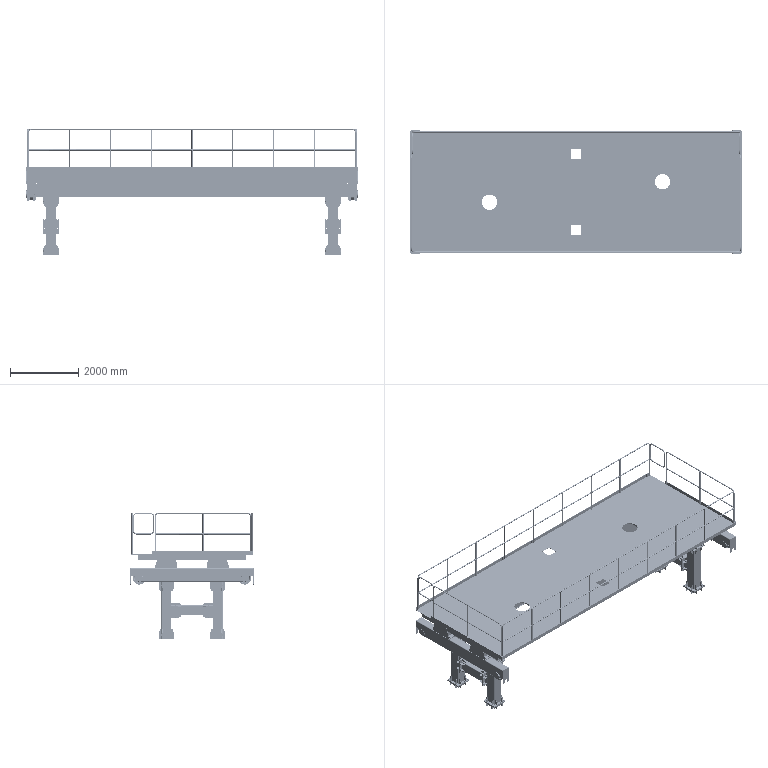Assembly | SolidWorks | mm | 353 component files | 557 solids | 9634 faces | box 9711 x 3600 x 3701.75 mm | volume 1285155719 mm3 | plane 4450 | cylinder 3136 | cone 1736 | torus 312 | commonest cylinder face diameters 21 x576 11 x384 12 x240 25 x192 20 x160 13 x144 24 x144 30 x128
Bill of materials:
Block | 24 | Plain Carbon Steel | Thin, flat square plate with rounded corners and no holes.
CrossRib | 2 |  | Multi-body fabricated frame: a long square hollow section with a bolted plate frame at each end, tapered gusset plates and protruding fin plates.
Door | 2 | Plain Carbon Steel | Closed loop of round-section rod or wire shaped as a square with large-radius rounded corners.
Flange10 | 4 | Plain Carbon Steel | Thin rectangular flat plate with sharp corners and two pairs of through-holes, one pair near each short end.
Flange20 | 4 | Plain Carbon Steel | Rectangular flat plate with sharp corners and a column of four through-holes along each short edge, eight holes in total.
GuardrailMountingPlate | 24 | Plain Carbon Steel | Thick rectangular plate with sharp corners and four through-holes, one near each corner.
Kick1 | 2 | Plain Carbon Steel | Very thin, flat rectangular sheet or strip that looks almost like a line in several views.
Kick2 | 2 | Plain Carbon Steel | Long, slender flat bar with small through-holes in groups of four at each end and at mid-length.
Link1 | 12 | Plain Carbon Steel | Long square hollow section with rounded corners and open ends. There is a slight offset or step at the ends.
Link2 | 24 | Plain Carbon Steel | Square hollow section with rounded corners and open ends, shorter relative to its cross-section than the similar tube body. There is a slight step at the ends.
350X125X10 | 8 | Plain Carbon Steel | Flat plate with a tapered profile, like a gusset: one long straight edge, one sloped edge, and a short straight section at the wide end.
650X450X360X10 | 4 | Plain Carbon Steel | Thin flat plate with a symmetric trapezoidal profile and short straight edges on each side at the wide base.
750X388X6 | 26 | Plain Carbon Steel | Thin flat rectangular plate with two narrow straight slots, one cut in from each long edge at about mid-height.
9340X450X10 | 2 | Plain Carbon Steel | Long, narrow, thin flat rectangular strip with no visible holes or features.
9340X60X6 | 4 | Plain Carbon Steel | Long, slender flat bar or strip with a thin rectangular cross-section and no visible features.
9940X450X10 | 2 | Plain Carbon Steel | Long, narrow, thin flat rectangular strip with no visible holes or features.
9940X9340X750X6 | 4 | Plain Carbon Steel | Long, thin flat bar with a stepped profile: a full-length upper band over a slightly shorter lower band, which leaves a shoulder notch at each end.
L | 4 | Plain Carbon Steel | Sheet bracket bent to a 90-degree L with a rounded inside bend. Both flanges have round through-holes near their ends.
Platform | 1 | Plain Carbon Steel | Very thin flat rectangular plate with two round holes and two small square holes.
PlatformGuardrail1 | 2 | Plain Carbon Steel | Slender round rod or wire bent into a wide U (staple-like shape) with rounded bends and two short parallel legs.
PlatformGuardrail2 | 16 | Plain Carbon Steel | Straight hollow round tube with plain cut ends.
PlatformGuardrail3 | 2 | Plain Carbon Steel | Long, slender straight hollow round tube with small evenly spaced marks along its length.
PlatformGuardrail4 | 2 | Plain Carbon Steel | Round rod or tube bent into a U shape with rounded bends and two longer parallel legs.
PlatformGuardrail5 | 2 | Plain Carbon Steel | Straight hollow round tube with a small circumferential groove or break at mid-length.
50 x 30 x 2.6x250 | 2 | Plain Carbon Steel | Long, straight, thin-walled hollow profile. The cross-section looks like a rectangle with rounded corners. Near each end, one side of the profile is cut back so the end sections are open channels (U-shaped). There is a rounded, roughly semicircular notch at each place where the cut-back ends meet the full-depth middle section.
380X230X6 | 8 | Plain Carbon Steel | Thin flat rectangular plate with four rounded corners and no visible holes or cutouts.
Finishing | 4 | Plain Carbon Steel | Thin flat rectangular plate with rounded outer corners, five round through-holes and a rectangular notch open to one short edge.
L756AngleBoxSingleEdgeWheelSet350-C | 4 |  | Axisymmetric wheel-like body with a single flange on one side. A short cylindrical housing projects from each face and has a ring of hex-head fasteners and a small central nipple-like protrusion.
100X75X8 | 64 | Plain Carbon Steel | Solid rectangular block (thick plate) with sharp edges and no visible features.
150X75X8 | 64 | Plain Carbon Steel | Flat plate of uniform thickness with an irregular five-sided outline: two parallel vertical edges of different heights, a short flat top, a long angled edge and a straight bottom edge.
300 x 300 x 8-100 | 8 | Plain Carbon Steel | Short, thin-walled square tube section (open frame ring) with rounded outer and inner corners, open at both ends.
300 x 300 x 8-1200 | 4 | Plain Carbon Steel | Long, thin-walled square hollow tube with rounded corners and open, square-cut ends.
450X450X20 | 16 | Plain Carbon Steel | Thin flat square plate with rounded corners and twelve round through-holes evenly spaced around the edge, four per side including the corners.
Mates:
1. coincident | Main-1/9940X450X10-1 face at (-3372.199, 2146.323, 5575.973) dir (0, 0, 1) | Platform-1 face at (1462.801, 1171.323, 5575.973) dir (0, 0, -1)
2. coincident | Main-2/650X450X360X10-2 face at (6307.801, 746.323, 5575.973) dir (1, 0, 0) | Platform-1 face at (6307.801, 2961.323, 5575.973) dir (1, 0, 0)
3. coincident | Platform-1 edge at (-3382.199, 1171.323, 5575.973) dir (1, 0, 0) | assembly plane at (0, 1171.323, 0) dir (0, -1, 0)
4. coincident | Main-1/L-1 face at (-3392.199, 1596.323, 5195.973) dir (0, 0, -1) | Flange10-1 face at (-3392.199, 1596.323, 5195.973) dir (0, 0, 1)
5. concentric | Main-1/L-1 face at (-3307.199, 2196.323, 4795.973) dir (0, 0, 1) r 12.5 | Flange10-1 face at (-3307.199, 2196.323, 4775.973) dir (0, 0, 1) r 12.5
6. concentric | Main-1/L-1 face at (-3307.199, 1646.323, 4795.973) dir (0, 0, 1) r 12.5 | Flange10-1 face at (-3307.199, 1646.323, 4775.973) dir (0, 0, 1) r 12.5
7. coincident | Main-1/L-1 face at (-3092.199, 1596.323, 5215.973) dir (-1, 0, 0) | Flange20-1 face at (-3092.199, 2246.323, 5215.973) dir (1, 0, 0)
8. concentric | Main-1/L-1 face at (-3392.199, 2196.323, 4870.973) dir (1, 0, 0) r 12.5 | Flange20-1 face at (-2792.199, 2196.323, 4870.973) dir (-1, 0, 0) r 12.5
9. concentric | Main-1/L-1 face at (-3392.199, 1646.323, 5140.973) dir (1, 0, 0) r 12.5 | Flange20-1 face at (-2792.199, 1646.323, 5140.973) dir (-1, 0, 0) r 12.5
10. coincident | Flange20-2 face at (-3112.199, 746.323, 5215.973) dir (-1, 0, 0) | Short-1/3650-1 face at (-3112.199, -618.677, 5165.973) dir (1, 0, 0)
11. coincident | Flange10-1 face at (-3392.199, 1596.323, 5185.973) dir (0, 0, -1) | Short-1/3650-1 face at (-3132.199, -618.677, 5185.973) dir (0, 0, 1)
12. coincident | Short-1 plane at (-2112.199, 1171.323, 4760.606) dir (0, 1, 0) | assembly plane at (0, 1171.323, 0) dir (0, -1, 0)
13. coincident | Flange20-4 face at (6037.801, 746.323, 5215.973) dir (1, 0, 0) | Short-3/3650-1 face at (6037.801, 2961.323, 5165.973) dir (-1, 0, 0)
14. coincident | Flange10-4 face at (6317.801, 746.323, 5185.973) dir (0, 0, -1) | Short-3/3650-1 face at (6057.801, 2961.323, 5185.973) dir (0, 0, 1)
15. coincident | Short-1/Finishing-1 face at (-3197.199, -628.677, 4795.973) dir (0, -1, 0) | Short-3/Finishing-2 face at (6202.801, -628.677, 4795.973) dir (0, -1, 0)
16. coincident | Main-1/9340X450X10-1 face at (-3072.199, 2146.323, 4805.973) dir (0, 0, -1) | TrolleyLeg-1/300 x 300 x 8-100-1 face at (-2796.199, 2055.323, 4805.973) dir (0, 0, 1)
17. coincident | Main-1/9340X450X10-1 face at (-3072.199, 2146.323, 4805.973) dir (0, 1, 0) | TrolleyLeg-1/450X450X20-3 face at (-2872.199, 2146.323, 4685.973) dir (0, 1, 0)
18. distance | assembly plane at (1462.801, 0, 0) dir (-1, 0, 0) | TrolleyLeg-1/300 x 300 x 8-100-1 edge at (-2662.199, 2071.323, 4805.973) dir (1, 0, 0)
19. coincident | TrolleyLeg-2/300 x 300 x 8-1200-1 face at (5737.801, 1787.323, 3245.973) dir (1, 0, 0) | CrossRib-1 face at (5737.801, 711.323, 4089.973) dir (1, 0, 0)
20. coincident | TrolleyLeg-2/300 x 300 x 8-1200-1 face at (5721.801, 1771.323, 3245.973) dir (0, -1, 0) | CrossRib-1 face at (5453.801, 1771.323, 3821.973) dir (0, 1, 0)
21. distance | CrossRib-1 face at (5453.801, 711.323, 3805.973) dir (0, 0, -1) | TrolleyLeg-2/300 x 300 x 8-100-2 face at (5721.801, 1787.323, 3105.973) dir (0, 0, -1)
22. coincident | Platform-1 face at (1462.801, 1171.323, 5585.973) dir (0, 0, 1) | Kick1-1 face at (-3382.199, 2951.323, 5585.973) dir (0, 0, -1)
23. parallel | Platform-1 face at (-3382.199, 2961.323, 5575.973) dir (0, 1, 0) | Kick1-1 face at (-3382.199, 2961.323, 5585.973) dir (0, 1, 0)
24. coincident | Platform-1 face at (6307.801, 2961.323, 5575.973) dir (1, 0, 0) | Kick1-1 face at (6307.801, 2951.323, 5585.973) dir (1, 0, 0)
25. coincident | Platform-1 face at (1462.801, 1171.323, 5585.973) dir (0, 0, 1) | Kick2-1 face at (6307.801, -608.677, 5585.973) dir (0, 0, -1)
26. distance | Kick1-1 face at (-3382.199, 2951.323, 5585.973) dir (0, -1, 0) | Platform-1 face at (-3382.199, 2961.323, 5575.973) dir (0, 1, 0)
27. coincident | Platform-1 face at (6307.801, 2961.323, 5575.973) dir (1, 0, 0) | Kick2-1 face at (6307.801, -608.677, 5585.973) dir (1, 0, 0)
28. coincident | Platform-1 face at (1462.801, 1171.323, 5575.973) dir (0, 0, -1) | Link1-1 face at (4455.801, 621.323, 5575.973) dir (0, 0, 1)
29. coincident | Main-2/9940X9340X750X6-1 face at (-3372.199, 621.323, 5565.973) dir (0, 1, 0) | Link1-1 face at (4455.801, 621.323, 5563.973) dir (0, -1, 0)
30. distance | Link1-1 face at (4317.801, 621.323, 5437.973) dir (-1, 0, 0) | Platform-1 face at (3992.801, 1471.323, 5575.973) dir (0, 0, 1) r 225
31. coincident | Main-2/9940X9340X750X6-2 face at (-3372.199, 221.323, 5565.973) dir (0, -1, 0) | Link2-1 edge at (4467.801, 221.323, 5563.973) dir (0, 0, -1)
32. coincident | Platform-1 face at (1462.801, 1171.323, 5575.973) dir (0, 0, -1) | Link2-1 face at (4455.801, -393.677, 5575.973) dir (0, 0, 1)
33. coincident | Link1-1 face at (4467.801, 621.323, 5563.973) dir (1, 0, 0) | Link2-1 face at (4467.801, -393.677, 5563.973) dir (1, 0, 0)
34. coincident | Platform-1 face at (1462.801, 1171.323, 5575.973) dir (0, 0, -1) | Link2-13 face at (4329.801, 2736.323, 5575.973) dir (0, 0, 1)
35. coincident | Main-1/9940X9340X750X6-1 face at (-3372.199, 2121.323, 5565.973) dir (0, 1, 0) | Link2-13 edge at (4467.801, 2121.323, 5500.973) dir (1, 0, 0)
36. coincident | Link1-1 face at (4317.801, 621.323, 5437.973) dir (-1, 0, 0) | Link2-13 face at (4317.801, 2736.323, 5563.973) dir (-1, 0, 0)
37. coincident | Link2-13 face at (4329.801, 2736.323, 5563.973) dir (0, 1, 0) | Block-1 face at (4333.801, 2736.323, 5559.973) dir (0, 1, 0)
38. coincident | Link2-13 face at (4461.801, 2736.323, 5437.973) dir (-1, 0, 0) | Block-1 face at (4461.801, 2730.323, 5441.973) dir (1, 0, 0)
39. coincident | Link2-13 face at (4455.801, 2736.323, 5431.973) dir (0, 0, 1) | Block-1 face at (4333.801, 2730.323, 5431.973) dir (0, 0, -1)
40. coincident | Link2-1 face at (4455.801, -393.677, 5563.973) dir (0, -1, 0) | Block-15 face at (4333.801, -393.677, 5559.973) dir (0, -1, 0)
41. coincident | Link2-1 face at (4323.801, -393.677, 5437.973) dir (1, 0, 0) | Block-15 face at (4323.801, -393.677, 5441.973) dir (-1, 0, 0)
42. coincident | Link2-1 face at (4329.801, -393.677, 5431.973) dir (0, 0, 1) | Block-15 face at (4333.801, -393.677, 5431.973) dir (0, 0, -1)
43. distance | Platform-1 face at (1462.801, 1171.323, 5585.973) dir (0, 0, 1) | PlatformGuardrail1-1 face at (-3322.199, -581.927, 5590.973) dir (0, 0, -1)
44. coincident | Kick1-2 face at (-3382.199, -608.677, 5685.973) dir (0, 1, 0) | GuardrailMountingPlate-1 face at (-3372.199, -608.677, 5585.973) dir (0, -1, 0)
45. coincident | Platform-1 face at (1462.801, 1171.323, 5585.973) dir (0, 0, 1) | GuardrailMountingPlate-1 face at (-3372.199, -608.677, 5585.973) dir (0, 0, -1)
46. coincident | Kick2-2 face at (-3372.199, -608.677, 5685.973) dir (1, 0, 0) | GuardrailMountingPlate-1 face at (-3372.199, -608.677, 5585.973) dir (-1, 0, 0)
47. distance | PlatformGuardrail1-1 face at (-3322.199, -581.927, 6690.973) dir (0, 0, -1) r 13.75 | GuardrailMountingPlate-1 face at (-3372.199, -598.677, 5585.973) dir (0, 1, 0)
48. distance | PlatformGuardrail1-1 face at (-3322.199, -581.927, 6690.973) dir (0, 0, -1) r 13.75 | GuardrailMountingPlate-1 face at (-3372.199, -608.677, 5585.973) dir (-1, 0, 0)
49. distance | GuardrailMountingPlate-1 face at (-3372.199, -598.677, 5585.973) dir (0, 1, 0) | PlatformGuardrail1-1 face at (6247.801, -581.927, 5590.973) dir (0, 0, 1) r 13.75
50. distance | PlatformGuardrail2-1 face at (-2110.949, -581.927, 6774.223) dir (0, 0, -1) r 16.75 | GuardrailMountingPlate-2 face at (-2180.949, -598.677, 5585.973) dir (0, 1, 0)
51. distance | GuardrailMountingPlate-2 face at (-2180.949, -608.677, 5585.973) dir (-1, 0, 0) | PlatformGuardrail2-1 face at (-2110.949, -581.927, 6774.223) dir (0, 0, -1) r 16.75
52. distance | PlatformGuardrail2-1 face at (-2110.949, -581.927, 6774.223) dir (0, 0, 1) | PlatformGuardrail1-1 face at (6147.801, -581.927, 6790.973) dir (-1, 0, 0) r 13.75
53. distance | Platform-1 face at (1462.801, 1171.323, 5585.973) dir (0, 0, 1) | PlatformGuardrail3-1 face at (-3305.449, -581.927, 6185.973) dir (1, 0, 0) r 16.75
54. distance | GuardrailMountingPlate-2 face at (-2180.949, -598.677, 5585.973) dir (0, 1, 0) | PlatformGuardrail3-1 face at (-3305.449, -581.927, 6185.973) dir (1, 0, 0) r 16.75
55. distance | PlatformGuardrail1-1 face at (-3322.199, -581.927, 6690.973) dir (0, 0, -1) r 13.75 | PlatformGuardrail3-1 face at (-3305.449, -581.927, 6185.973) dir (-1, 0, 0)
56. coincident | Kick2-1 face at (6297.801, -608.677, 5585.973) dir (-1, 0, 0) | GuardrailMountingPlate-19 face at (6297.801, -598.677, 5585.973) dir (1, 0, 0)
57. coincident | Kick2-1 face at (6307.801, -608.677, 5685.973) dir (0, 0, 1) | GuardrailMountingPlate-19 face at (6297.801, -598.677, 5685.973) dir (0, 0, 1)
58. coincident | GuardrailMountingPlate-9 face at (6157.801, -598.677, 5585.973) dir (0, 1, 0) | GuardrailMountingPlate-19 face at (6297.801, -598.677, 5585.973) dir (0, -1, 0)
59. distance | PlatformGuardrail4-1 face at (6271.051, -551.927, 5590.973) dir (0, 0, -1) | Platform-1 face at (1462.801, 1171.323, 5585.973) dir (0, 0, 1)
60. distance | GuardrailMountingPlate-19 face at (6287.801, -598.677, 5585.973) dir (-1, 0, 0) | PlatformGuardrail4-1 face at (6271.051, -551.927, 5590.973) dir (0, 0, 1) r 16.75
61. distance | PlatformGuardrail4-1 face at (6271.051, -551.927, 5590.973) dir (0, 0, 1) r 16.75 | Kick1-2 face at (-3382.199, -608.677, 5685.973) dir (0, 1, 0)
62. coincident | Kick2-1 face at (6297.801, -608.677, 5585.973) dir (-1, 0, 0) | GuardrailMountingPlate-20 face at (6297.801, 2194.823, 5585.973) dir (1, 0, 0)
63. coincident | Kick2-1 face at (6307.801, -608.677, 5685.973) dir (0, 0, 1) | GuardrailMountingPlate-20 face at (6297.801, 2194.823, 5685.973) dir (0, 0, 1)
64. distance | PlatformGuardrail4-1 face at (6271.051, 2248.073, 6690.973) dir (0, 0, -1) r 16.75 | GuardrailMountingPlate-20 face at (6297.801, 2334.823, 5585.973) dir (0, 1, 0)
65. distance | GuardrailMountingPlate-21 face at (6287.801, 794.823, 5585.973) dir (-1, 0, 0) | PlatformGuardrail2-15 face at (6271.051, 848.073, 6774.223) dir (0, 0, -1) r 16.75
66. coincident | PlatformGuardrail2-7 face at (5036.551, -581.927, 6774.223) dir (0, 0, 1) | PlatformGuardrail2-15 face at (6271.051, 848.073, 6774.223) dir (0, 0, 1)
67. distance | PlatformGuardrail2-15 face at (6271.051, 848.073, 6774.223) dir (0, 0, -1) r 16.75 | GuardrailMountingPlate-21 face at (6297.801, 934.823, 5585.973) dir (0, 1, 0)
68. distance | Platform-1 face at (1462.801, 1171.323, 5585.973) dir (0, 0, 1) | PlatformGuardrail5-1 face at (6271.051, 2224.823, 6185.973) dir (0, -1, 0) r 16.75
69. distance | GuardrailMountingPlate-21 face at (6287.801, 794.823, 5585.973) dir (-1, 0, 0) | PlatformGuardrail5-1 face at (6271.051, 2224.823, 6185.973) dir (0, -1, 0) r 16.75
70. distance | PlatformGuardrail4-1 face at (6271.051, -551.927, 5590.973) dir (0, 0, 1) r 16.75 | PlatformGuardrail5-1 face at (6271.051, -535.177, 6185.973) dir (0, -1, 0)
71. distance | Door-1 face at (6247.801, 2888.323, 6685.973) dir (0, 0, 1) r 16.75 | Kick2-1 face at (6297.801, -608.677, 5585.973) dir (-1, 0, 0)
72. distance | Door-1 face at (6247.801, 2888.323, 6685.973) dir (0, 0, 1) r 16.75 | Kick1-1 face at (-3382.199, 2961.323, 5585.973) dir (0, 1, 0)
73. distance | Door-1 face at (6247.801, 2788.323, 6185.973) dir (0, 1, 0) r 16.75 | Platform-1 face at (1462.801, 1171.323, 5585.973) dir (0, 0, 1)
74. coincident | 9940X450X10-1 face at (-6309.119, 904.191, 1000) dir (0, -1, 0) | 9940X9340X750X6-1 face at (-6309.119, 904.191, 1025) dir (0, 1, 0)
75. coincident | 9940X450X10-1 face at (-6309.119, 904.191, 1000) dir (-1, 0, 0) | 9940X9340X750X6-1 face at (-6309.119, 554.191, 1025) dir (-1, 0, 0)
76. distance | 9940X450X10-1 face at (-6309.119, 904.191, 1000) dir (0, 0, -1) | 9940X9340X750X6-1 face at (-6309.119, 904.191, 1025) dir (0, 0, -1)
77. coincident | 9940X9340X750X6-1 face at (-6309.119, 904.191, 1031) dir (0, 0, 1) | 750X388X6-1 face at (-5868.119, 154.191, 1031) dir (0, 0, -1)
78. coincident | 9940X450X10-1 face at (-6309.119, 904.191, 1000) dir (0, -1, 0) | 750X388X6-1 face at (-5868.119, 904.191, 1031) dir (0, 1, 0)
79. distance | 750X388X6-1 face at (-5874.119, 904.191, 1031) dir (-1, 0, 0) | 9940X9340X750X6-1 face at (-6009.119, 154.191, 1025) dir (-1, 0, 0)
80. coincident | 750X388X6-1 face at (-5868.119, 524.191, 1031) dir (0, 1, 0) | 9340X60X6-1 face at (-6009.119, 524.191, 1031) dir (0, -1, 0)
81. coincident | 9940X9340X750X6-1 face at (-6309.119, 904.191, 1031) dir (0, 0, 1) | 9340X60X6-1 face at (-6009.119, 524.191, 1031) dir (0, 0, -1)
82. coincident | 9940X9340X750X6-1 face at (-6009.119, 154.191, 1025) dir (-1, 0, 0) | 9340X60X6-1 face at (-6009.119, 524.191, 1031) dir (-1, 0, 0)
83. coincident | 750X388X6-1 face at (-5868.119, 524.191, 1354) dir (0, 1, 0) | 9340X60X6-2 face at (-6009.119, 524.191, 1359) dir (0, -1, 0)
84. coincident | 750X388X6-1 face at (-5868.119, 904.191, 1419) dir (0, 0, 1) | 9340X60X6-2 face at (-6009.119, 524.191, 1419) dir (0, 0, 1)
85. coincident | 9340X60X6-1 face at (-6009.119, 524.191, 1031) dir (-1, 0, 0) | 9340X60X6-2 face at (-6009.119, 524.191, 1359) dir (-1, 0, 0)
86. coincident | 750X388X6-1 face at (-5868.119, 154.191, 1419) dir (0, -1, 0) | 9340X450X10-1 face at (-6009.119, 154.191, 1000) dir (0, 1, 0)
87. coincident | 9940X450X10-1 face at (-6309.119, 904.191, 1000) dir (0, 0, -1) | 9340X450X10-1 face at (-6009.119, 144.191, 1000) dir (0, 0, -1)
88. coincident | 9940X9340X750X6-1 face at (-6009.119, 154.191, 1025) dir (-1, 0, 0) | 9340X450X10-1 face at (-6009.119, 144.191, 1000) dir (-1, 0, 0)
89. coincident | 750X388X6-1 face at (-5868.119, 524.191, 1419) dir (0, 0, 1) | 9940X9340X750X6-2 face at (-6309.119, 904.191, 1419) dir (0, 0, -1)
90. coincident | 9940X450X10-1 face at (-6309.119, 904.191, 1000) dir (0, -1, 0) | 9940X9340X750X6-2 face at (-6309.119, 904.191, 1419) dir (0, 1, 0)
91. coincident | 9940X450X10-1 face at (-6309.119, 904.191, 1000) dir (-1, 0, 0) | 9940X9340X750X6-2 face at (-6309.119, 554.191, 1419) dir (-1, 0, 0)
92. coincident | 9940X9340X750X6-2 face at (-6009.119, 154.191, 1419) dir (-1, 0, 0) | L-1 face at (-6009.119, 554.191, 1550) dir (1, 0, 0)
93. coincident | 9940X9340X750X6-2 face at (-6009.119, 554.191, 1419) dir (0, -1, 0) | L-1 face at (-6329.119, 554.191, 1550) dir (0, 1, 0)
94. distance | 9940X9340X750X6-1 face at (-6309.119, 904.191, 1025) dir (0, 0, -1) | L-1 face at (-6029.119, 509.191, 900) dir (0, 0, -1)
95. coincident | 9940X9340X750X6-2 face at (-6309.119, 554.191, 1419) dir (-1, 0, 0) | 650X450X360X10-1 face at (-6309.119, 914.191, 1550) dir (1, 0, 0)
96. coincident | L-1 face at (-6329.119, 554.191, 1550) dir (0, 1, 0) | 650X450X360X10-1 face at (-6319.119, 554.191, 900) dir (0, -1, 0)
97. coincident | L-1 face at (-6054.119, 509.191, 1550) dir (0, 0, 1) | 650X450X360X10-1 face at (-6319.119, 554.191, 1550) dir (0, 0, 1)
98. coincident | L-1 face at (-6054.119, 509.191, 1550) dir (0, 0, 1) | 350X125X10-1 face at (-6054.119, 604.191, 1550) dir (0, 0, 1)
99. coincident | L-1 edge at (-6054.119, 554.191, 1550) dir (0, 0, -1) | 350X125X10-1 edge at (-6054.119, 554.191, 1425) dir (0, 0, 1)
100. coincident | L-1 face at (-6329.119, 554.191, 1550) dir (0, 1, 0) | 350X125X10-1 face at (-6054.119, 554.191, 1550) dir (0, -1, 0)
101. coincident | L-1 face at (-6029.119, 509.191, 900) dir (0, 0, -1) | 350X125X10-2 face at (-6064.119, 604.191, 900) dir (0, 0, -1)
102. coincident | L-1 edge at (-6054.119, 554.191, 1550) dir (0, 0, -1) | 350X125X10-2 face at (-6064.119, 554.191, 900) dir (0, -1, 0)
103. coincident | L-1 edge at (-6054.119, 554.191, 1550) dir (0, 0, -1) | 350X125X10-2 face at (-6054.119, 904.191, 1025) dir (1, 0, 0)
104. coincident | L-1 face at (-6329.119, 554.191, 1550) dir (0, 1, 0) | 350X125X10-2 face at (-6064.119, 554.191, 900) dir (0, -1, 0)
105. distance | 380X230X6-1 face at (-3007.575, 400.367, 1025) dir (-1, 0, 0) | 3650-1 face at (-3622.575, 45.367, 1230) dir (-1, 0, 0)
106. coincident | 3650-1 face at (-42.575, 415.367, 1020) dir (0, -1, 0) | 380X230X6-1 face at (-2997.575, 415.367, 1025) dir (0, 1, 0)
107. coincident | 3650-1 face at (-42.575, 405.367, 1010) dir (0, 0, 1) | 380X230X6-1 face at (-2997.575, 50.367, 1010) dir (0, 0, -1)
108. concentric | 3650-1 face at (-3372.575, 135.367, 1250) dir (0, 0, -1) r 105 | L756AngleBoxSingleEdgeWheelSet350-C-3 face at (-3372.575, 135.367, 1060) dir (0, 0, -1) r 105
109. distance | L756AngleBoxSingleEdgeWheelSet350-C-3 face at (-3402.058, 209.737, 979.5) dir (0, 0, -1) | 3650-1 face at (-42.575, 405.367, 1000) dir (0, 0, -1)
110. concentric | 3650-1 face at (-292.575, 135.367, 1250) dir (0, 0, -1) r 105 | L756AngleBoxSingleEdgeWheelSet350-C-4 face at (-292.575, 135.367, 1060) dir (0, 0, -1) r 105
111. distance | L756AngleBoxSingleEdgeWheelSet350-C-4 face at (-322.058, 209.737, 979.5) dir (0, 0, -1) | 3650-1 face at (-42.575, 405.367, 1000) dir (0, 0, -1)
112. coincident | 3650-1 face at (-42.575, 45.367, 1230) dir (1, 0, 0) | Finishing-1 face at (-42.575, 35.367, 1085) dir (-1, 0, 0)
113. coincident | 3650-1 face at (-42.575, 45.367, 1250) dir (0, 0, 1) | Finishing-1 face at (-32.575, 415.367, 1250) dir (0, 0, 1)
114. coincident | 3650-1 face at (-42.575, 425.367, 1020) dir (0, 1, 0) | Finishing-1 face at (-32.575, 425.367, 1010) dir (0, 1, 0)
115. coincident | 450X450X20-1 face at (1257.496, 982.157, 1230.34) dir (0, 1, 0) | 300 x 300 x 8-1200-1 face at (913.496, 982.157, 1306.34) dir (0, -1, 0)
116. distance | 300 x 300 x 8-1200-1 face at (897.496, 982.157, 1306.34) dir (-1, 0, 0) | 450X450X20-1 face at (822.496, 962.157, 1230.34) dir (-1, 0, 0)
117. distance | 300 x 300 x 8-1200-1 face at (913.496, 982.157, 1290.34) dir (0, 0, -1) | 450X450X20-1 face at (837.496, 962.157, 1215.34) dir (0, 0, -1)
118. coincident | 300 x 300 x 8-1200-1 face at (913.496, 2402.157, 1306.34) dir (0, 1, 0) | 450X450X20-2 face at (1257.496, 2402.157, 1230.34) dir (0, -1, 0)
119. distance | 300 x 300 x 8-1200-1 face at (913.496, 982.157, 1290.34) dir (0, 0, -1) | 450X450X20-2 face at (837.496, 2402.157, 1215.34) dir (0, 0, -1)
120. distance | 450X450X20-2 face at (822.496, 2402.157, 1230.34) dir (-1, 0, 0) | 300 x 300 x 8-1200-1 face at (897.496, 982.157, 1306.34) dir (-1, 0, 0)
121. coincident | 450X450X20-2 face at (1257.496, 2422.157, 1230.34) dir (0, 1, 0) | 450X450X20-3 face at (1257.496, 2422.157, 1230.34) dir (0, -1, 0)
122. concentric | 450X450X20-2 face at (852.496, 2402.157, 1635.34) dir (0, 1, 0) r 10.5 | 450X450X20-3 face at (852.496, 2422.157, 1635.34) dir (0, 1, 0) r 10.5
123. concentric | 450X450X20-2 face at (1242.496, 2402.157, 1245.34) dir (0, 1, 0) r 10.5 | 450X450X20-3 face at (1242.496, 2422.157, 1245.34) dir (0, 1, 0) r 10.5
124. coincident | 450X450X20-3 face at (1257.496, 2442.157, 1230.34) dir (0, 1, 0) | 300 x 300 x 8-100-1 face at (913.496, 2442.157, 1306.34) dir (0, -1, 0)
125. coincident | 300 x 300 x 8-1200-1 face at (897.496, 982.157, 1306.34) dir (-1, 0, 0) | 300 x 300 x 8-100-1 face at (897.496, 2442.157, 1306.34) dir (-1, 0, 0)
126. coincident | 300 x 300 x 8-1200-1 face at (913.496, 982.157, 1290.34) dir (0, 0, -1) | 300 x 300 x 8-100-1 face at (913.496, 2442.157, 1290.34) dir (0, 0, -1)
127. coincident | 300 x 300 x 8-100-1 face at (897.496, 2442.157, 1306.34) dir (-1, 0, 0) | 100X75X8-1 face at (897.496, 2542.157, 1326.34) dir (1, 0, 0)
128. coincident | 300 x 300 x 8-100-1 face at (913.496, 2542.157, 1306.34) dir (0, 1, 0) | 100X75X8-1 face at (822.496, 2542.157, 1326.34) dir (0, 1, 0)
129. distance | 450X450X20-3 face at (837.496, 2422.157, 1215.34) dir (0, 0, -1) | 100X75X8-1 face at (822.496, 2542.157, 1326.34) dir (0, 0, -1)
130. coincident | 300 x 300 x 8-100-1 face at (897.496, 2442.157, 1306.34) dir (-1, 0, 0) | 100X75X8-2 face at (897.496, 2542.157, 1544.34) dir (1, 0, 0)
131. coincident | 300 x 300 x 8-100-1 face at (913.496, 2542.157, 1306.34) dir (0, 1, 0) | 100X75X8-2 face at (822.496, 2542.157, 1544.34) dir (0, 1, 0)
132. distance | 300 x 300 x 8-100-1 face at (1181.496, 2442.157, 1590.34) dir (0, 0, 1) | 100X75X8-2 face at (822.496, 2542.157, 1554.34) dir (0, 0, 1)
133. coincident | 450X450X20-3 face at (837.496, 2422.157, 1665.34) dir (0, 0, 1) | 100X75X8-3 face at (933.496, 2542.157, 1665.34) dir (0, 0, 1)
134. coincident | 300 x 300 x 8-100-1 face at (913.496, 2542.157, 1306.34) dir (0, 1, 0) | 100X75X8-3 face at (933.496, 2542.157, 1665.34) dir (0, 1, 0)
135. distance | 300 x 300 x 8-100-1 face at (897.496, 2442.157, 1306.34) dir (-1, 0, 0) | 100X75X8-3 face at (933.496, 2542.157, 1665.34) dir (-1, 0, 0)
136. coincident | 300 x 300 x 8-100-1 face at (913.496, 2542.157, 1306.34) dir (0, 1, 0) | 100X75X8-4 face at (1151.496, 2542.157, 1665.34) dir (0, 1, 0)
137. coincident | 450X450X20-3 face at (837.496, 2422.157, 1665.34) dir (0, 0, 1) | 100X75X8-4 face at (1151.496, 2542.157, 1665.34) dir (0, 0, 1)
138. distance | 300 x 300 x 8-100-1 face at (1197.496, 2442.157, 1574.34) dir (1, 0, 0) | 100X75X8-4 face at (1161.496, 2542.157, 1665.34) dir (1, 0, 0)
139. coincident | 450X450X20-1 face at (1257.496, 982.157, 1230.34) dir (0, 1, 0) | 150X75X8-1 face at (1153.496, 982.157, 1215.34) dir (0, -1, 0)
140. coincident | 450X450X20-1 face at (837.496, 962.157, 1215.34) dir (0, 0, -1) | 150X75X8-1 face at (1153.496, 1032.157, 1215.34) dir (0, 0, -1)
141. distance | 300 x 300 x 8-1200-1 face at (1197.496, 982.157, 1574.34) dir (1, 0, 0) | 150X75X8-1 face at (1161.496, 1132.157, 1290.34) dir (1, 0, 0)
142. coincident | 450X450X20-1 face at (1257.496, 982.157, 1230.34) dir (0, 1, 0) | 150X75X8-2 face at (933.496, 982.157, 1215.34) dir (0, -1, 0)
143. coincident | 450X450X20-1 face at (837.496, 962.157, 1215.34) dir (0, 0, -1) | 150X75X8-2 face at (933.496, 1032.157, 1215.34) dir (0, 0, -1)
144. distance | 300 x 300 x 8-1200-1 face at (897.496, 982.157, 1306.34) dir (-1, 0, 0) | 150X75X8-2 face at (933.496, 1132.157, 1290.34) dir (-1, 0, 0)
145. coincident | 450X450X20-1 face at (1257.496, 982.157, 1230.34) dir (0, 1, 0) | 150X75X8-3 face at (1272.496, 982.157, 1326.34) dir (0, -1, 0)
146. coincident | 450X450X20-1 face at (1272.496, 962.157, 1230.34) dir (1, 0, 0) | 150X75X8-3 face at (1272.496, 1032.157, 1326.34) dir (1, 0, 0)
147. distance | 150X75X8-3 face at (1197.496, 1132.157, 1326.34) dir (0, 0, -1) | 300 x 300 x 8-1200-1 face at (913.496, 982.157, 1290.34) dir (0, 0, -1)
148. coincident | 450X450X20-1 face at (1257.496, 982.157, 1230.34) dir (0, 1, 0) | 150X75X8-4 face at (1272.496, 982.157, 1546.34) dir (0, -1, 0)
149. coincident | 450X450X20-1 face at (1272.496, 962.157, 1230.34) dir (1, 0, 0) | 150X75X8-4 face at (1272.496, 1032.157, 1546.34) dir (1, 0, 0)
150. distance | 300 x 300 x 8-1200-1 face at (1181.496, 982.157, 1590.34) dir (0, 0, 1) | 150X75X8-4 face at (1197.496, 1132.157, 1554.34) dir (0, 0, 1)